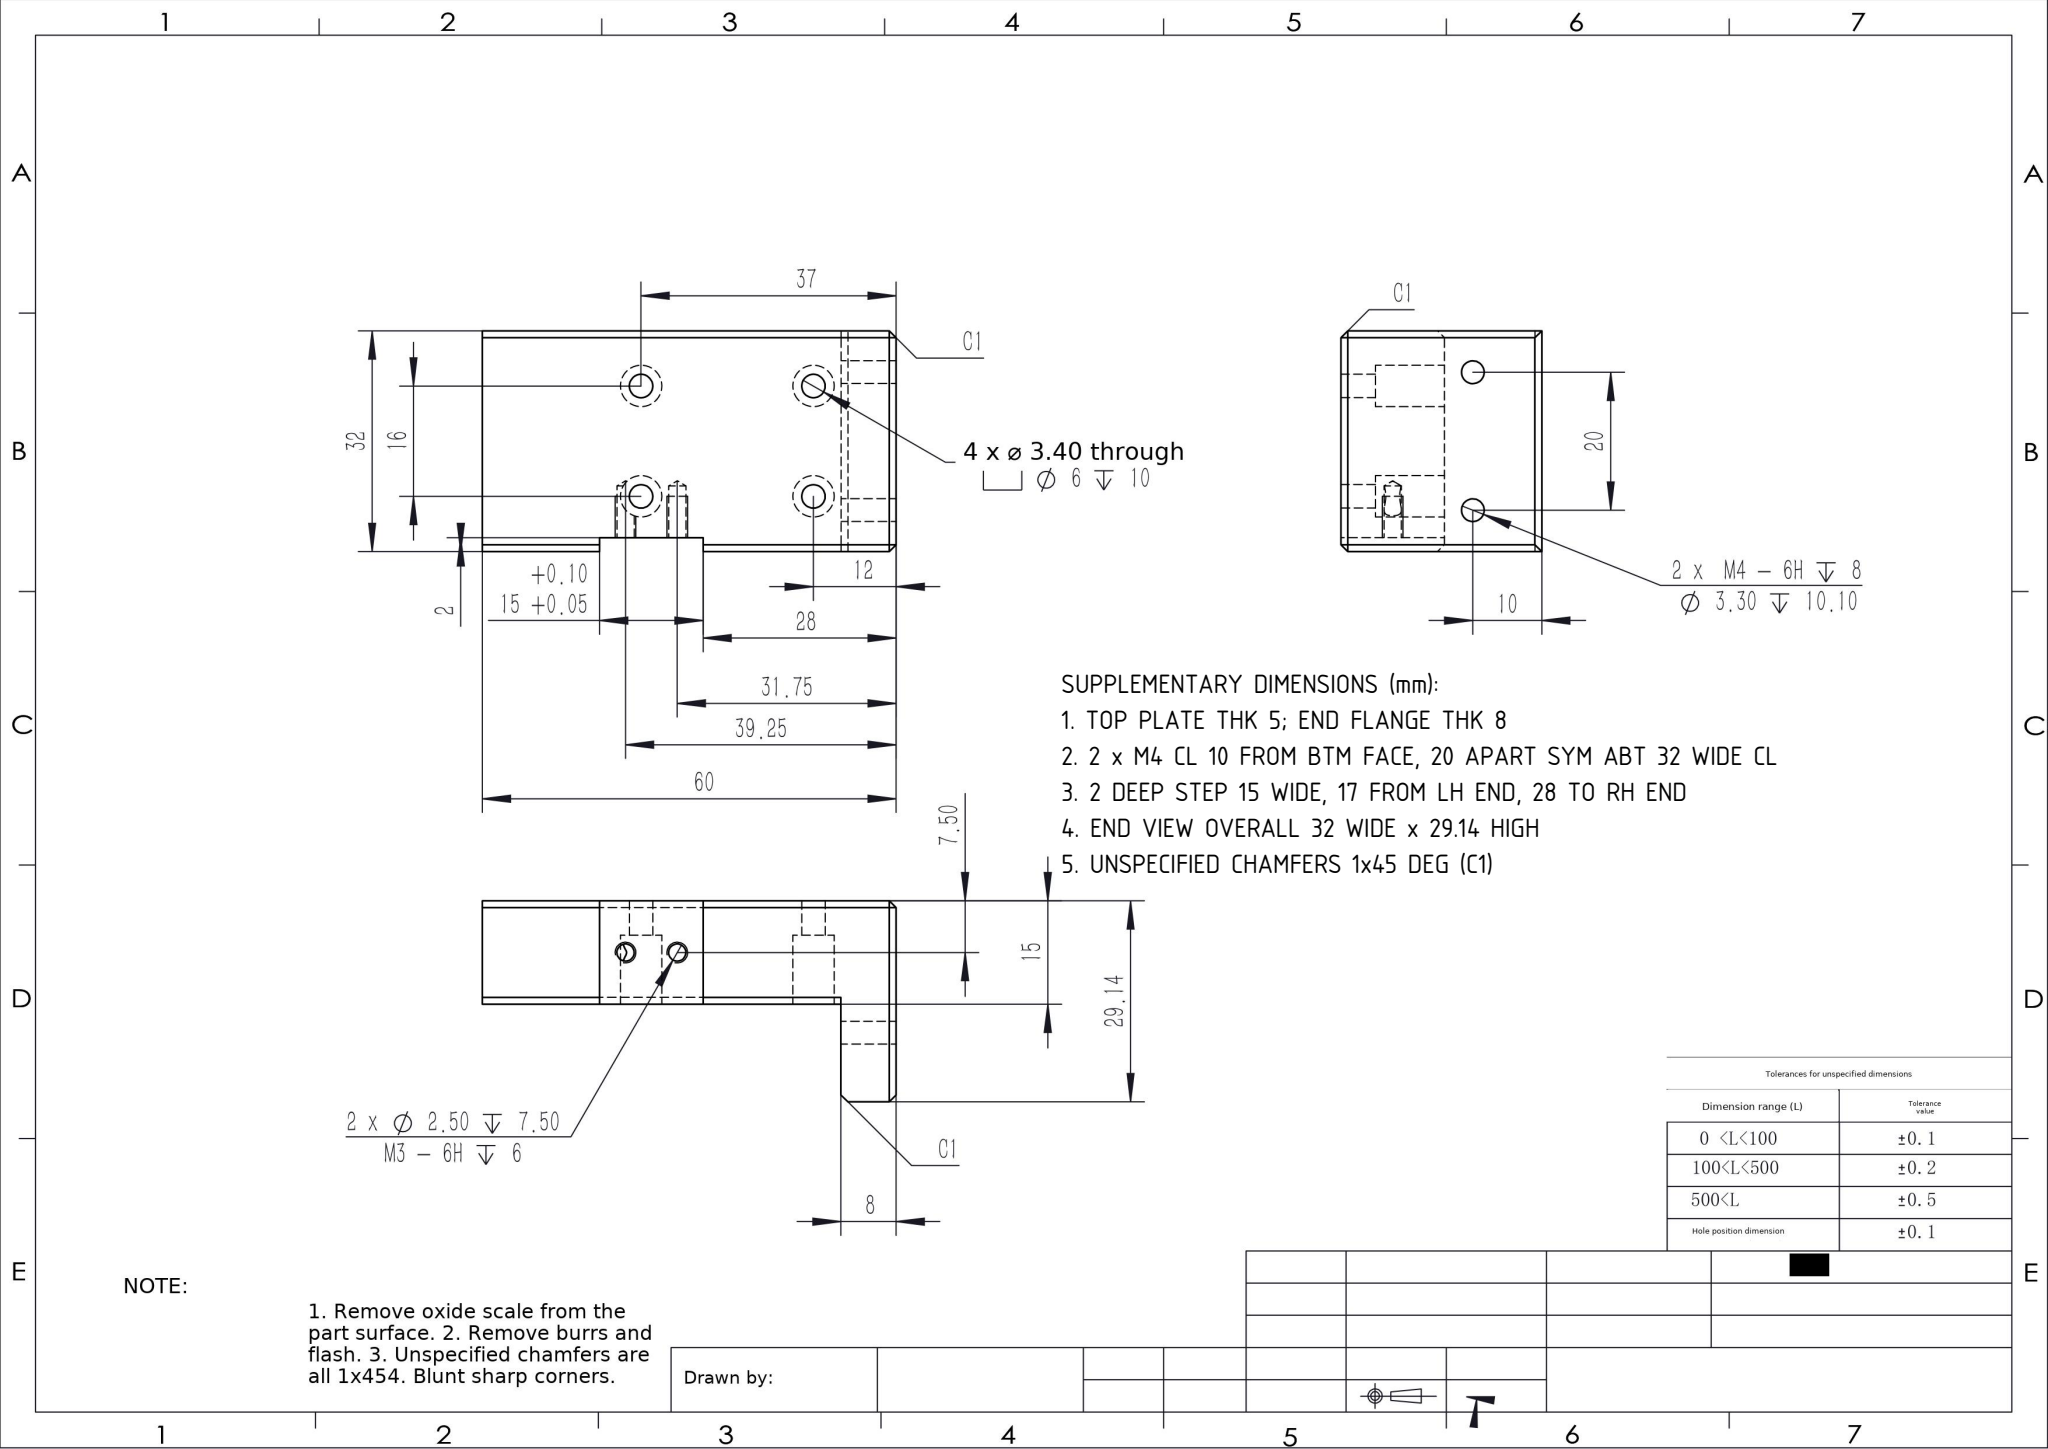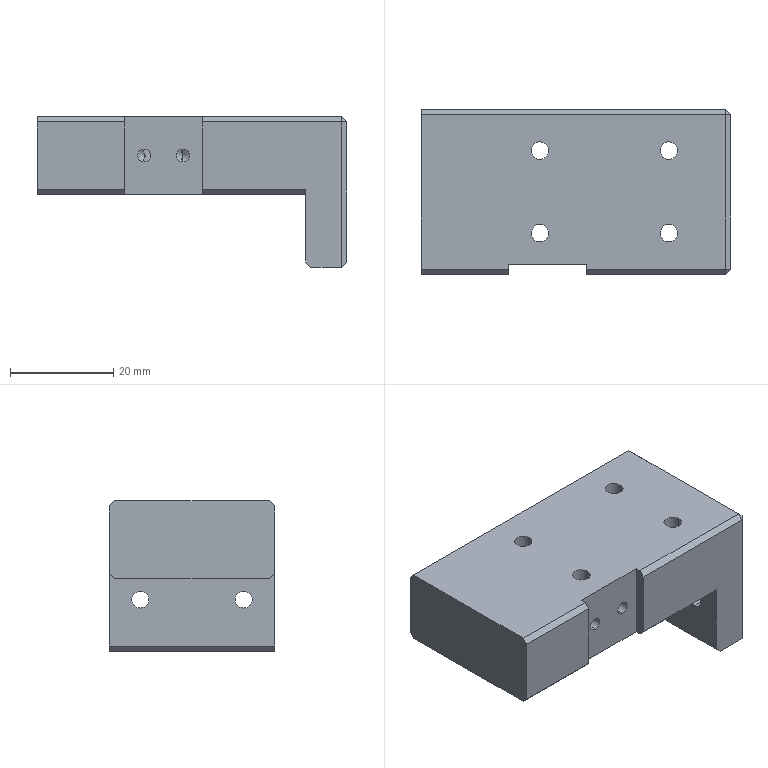Part | SolidWorks | mm | 1 solid | 57 faces | box 60 x 32 x 29.14 mm | volume 30286 mm3 | plane 29 | cylinder 24 | cone 4 | commonest cylinder face diameters 6 x8 3.4 x8 2.5 x4 3.3 x4
build123d program:
from build123d import *

# Parameters (mm, degrees)
SKETCH1_W                                            = 60
SKETCH1_H                                            = 32
BOSS_EXTRUDE1_DEPTH                                  = 15
SKETCH2_W                                            = 8
SKETCH2_H                                            = 32
BOSS_EXTRUDE2_DEPTH                                  = 14.136
HOLE_SIZE_ACCORDING_TO_THE_TYPE_OF_HEXAG_D           = 3.4
HOLE_SIZE_ACCORDING_TO_THE_TYPE_OF_HEXAG_CBORE_D     = 6
HOLE_SIZE_ACCORDING_TO_THE_TYPE_OF_HEXAG_CBORE_DEPTH = 10
M4_TAPPED_HOLE1_D                                    = 3.3
M4_TAPPED_HOLE1_DEPTH                                = 10.1
M4_TAPPED_HOLE1_TIP                                  = 0.9914
SKETCH7_W                                            = 15
SKETCH7_H                                            = 15
CUT_EXTRUDE1_DEPTH                                   = 2
CHAMFER1_SIZE                                        = 1
M3_TAPPED_HOLE1_D                                    = 2.5
M3_TAPPED_HOLE1_DEPTH                                = 7.5
M3_TAPPED_HOLE1_TIP                                  = 0.7511


with BuildPart() as part:
    # Sketch1 → Boss-Extrude1 (new body)
    with BuildSketch(Plane.XY):
        Rectangle(SKETCH1_W, SKETCH1_H)
    extrude(amount=BOSS_EXTRUDE1_DEPTH)

    # Sketch2 → Boss-Extrude2 (add)
    with BuildSketch(Plane(origin=(0, 0, 0), x_dir=(-1, 0, 0), z_dir=(0, 0, -1))):
        with Locations((-26, 0)):
            Rectangle(SKETCH2_W, SKETCH2_H)
    extrude(amount=BOSS_EXTRUDE2_DEPTH)

    # Hole Size according to the type of Hexag (through all)
    with Locations(Plane(origin=(0, 0, 0), x_dir=(-1, 0, 0), z_dir=(0, 0, -1))):
        with Locations((-18, 8), (-18, -8), (7, 8), (7, -8)):
            CounterBoreHole(HOLE_SIZE_ACCORDING_TO_THE_TYPE_OF_HEXAG_D / 2, HOLE_SIZE_ACCORDING_TO_THE_TYPE_OF_HEXAG_CBORE_D / 2, HOLE_SIZE_ACCORDING_TO_THE_TYPE_OF_HEXAG_CBORE_DEPTH)

    # M4 Tapped Hole1
    with Locations(Plane(origin=(30, 0, 0), x_dir=(0, 0, -1), z_dir=(1, 0, 0))):
        with Locations((4.136, 10), (4.136, -10)):
            Hole(M4_TAPPED_HOLE1_D / 2, depth=M4_TAPPED_HOLE1_DEPTH)
            with Locations((0, 0, -(M4_TAPPED_HOLE1_DEPTH + M4_TAPPED_HOLE1_TIP / 2))):  # 118° drill point
                Cone(0, M4_TAPPED_HOLE1_D / 2, M4_TAPPED_HOLE1_TIP, mode=Mode.SUBTRACT)

    # Sketch7 → Cut-Extrude1 (cut)
    with BuildSketch(Plane.XZ.offset(16)):
        with Locations((-5.5, 7.5)):
            Rectangle(SKETCH7_W, SKETCH7_H)
    extrude(amount=-CUT_EXTRUDE1_DEPTH, mode=Mode.SUBTRACT)

    # Chamfer1
    chamfer1_edges = [part.edges().sort_by_distance(p)[0] for p in [
        (-21.5, -16, 15),
        (-4, 16, 0),
        (30, 0, -14.136),
        (22, 0, -14.136),
        (30, 0, 15),
        (-21.5, -16, 0),
        (0, 16, 15),
        (16, -16, 15),
        (12, -16, 0),
        (30, -16, 0.4318),
        (30, 16, 0.4318),
    ]]
    chamfer(chamfer1_edges, length=CHAMFER1_SIZE)

    # M3 Tapped Hole1
    with Locations(Plane(origin=(0, -14, 0), x_dir=(-1, 0, 0), z_dir=(0, -1, 0))):
        with Locations((1.75, -7.5), (9.25, -7.5)):
            Hole(M3_TAPPED_HOLE1_D / 2, depth=M3_TAPPED_HOLE1_DEPTH)
            with Locations((0, 0, -(M3_TAPPED_HOLE1_DEPTH + M3_TAPPED_HOLE1_TIP / 2))):  # 118° drill point
                Cone(0, M3_TAPPED_HOLE1_D / 2, M3_TAPPED_HOLE1_TIP, mode=Mode.SUBTRACT)


solid = part.part